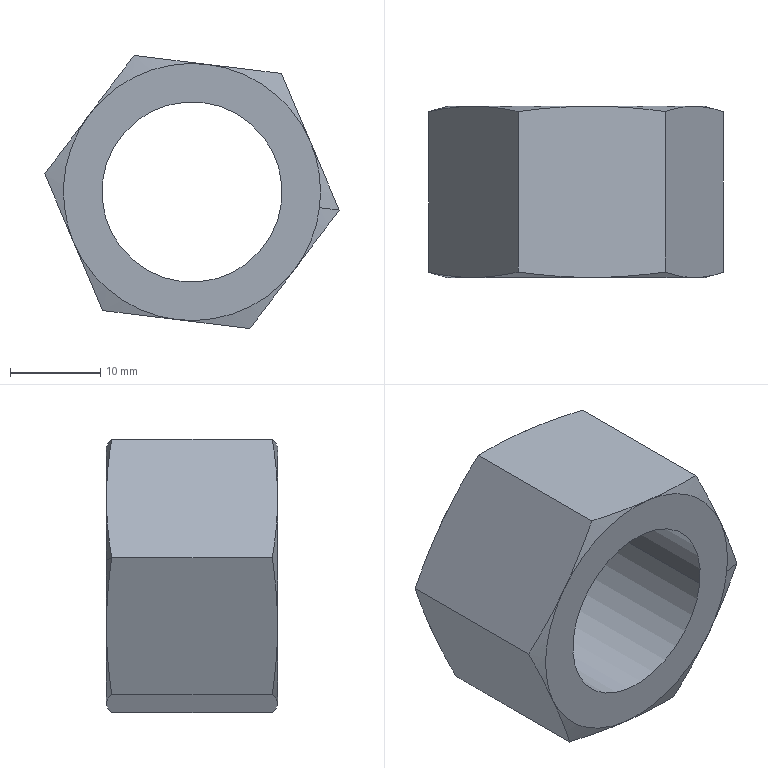Component | SolidWorks | GB_T41-2000HexNutType1C-gradeM20-1 | 1 solid | 24 faces | box 32.7 x 19 x 30.33 mm | volume 7406 mm3 | cone 14 | plane 8 | cylinder 2 | commonest cylinder face diameters 20 x2
STEP:
#1=COLOUR_RGB('',0.7922,0.8196,0.9333);
#2=FILL_AREA_STYLE_COLOUR('',#1);
#3=FILL_AREA_STYLE('',(#2));
#4=SURFACE_STYLE_FILL_AREA(#3);
#5=SURFACE_SIDE_STYLE('',(#4));
#6=SURFACE_STYLE_USAGE(.BOTH.,#5);
#7=PRESENTATION_STYLE_ASSIGNMENT((#6));
#8=CARTESIAN_POINT('',(-12.869,-7.053,5.337));
#9=VERTEX_POINT('',#8);
#10=CARTESIAN_POINT('',(-12.828,-7.053,5.05));
#11=VERTEX_POINT('',#10);
#12=CARTESIAN_POINT('',(-13.386,-7.053,5.118));
#13=DIRECTION('',(-0.,1.,0.));
#14=DIRECTION('',(-0.9925,0.,0.1221));
#15=AXIS2_PLACEMENT_3D('',#12,#13,#14);
#16=CIRCLE('',#15,0.5617);
#17=EDGE_CURVE('',#9,#11,#16,.T.);
#18=ORIENTED_EDGE('',*,*,#17,.T.);
#19=CARTESIAN_POINT('',(-12.742,-7.029,5.039));
#20=VERTEX_POINT('',#19);
#21=CARTESIAN_POINT('',(-12.828,-7.053,5.05));
#22=DIRECTION('',(0.9587,0.2588,-0.1179));
#23=VECTOR('',#22,39.37);
#24=LINE('',#21,#23);
#25=EDGE_CURVE('',#11,#20,#24,.T.);
#26=ORIENTED_EDGE('',*,*,#25,.T.);
#27=CARTESIAN_POINT('',(-12.742,-7.029,5.039));
#28=CARTESIAN_POINT('',(-12.763,-7.036,5.089));
#29=CARTESIAN_POINT('',(-12.784,-7.042,5.138));
#30=CARTESIAN_POINT('',(-12.826,-7.05,5.238));
#31=CARTESIAN_POINT('',(-12.848,-7.053,5.288));
#32=CARTESIAN_POINT('',(-12.869,-7.053,5.337));
#33=B_SPLINE_CURVE_WITH_KNOTS('',3,(#27,#28,#29,#30,#31,#32),.UNSPECIFIED.,.F.,.F.,(4,2,4),(0.00000023,0.004119,0.008238),.UNSPECIFIED.);
#34=EDGE_CURVE('',#20,#9,#33,.T.);
#35=ORIENTED_EDGE('',*,*,#34,.T.);
#36=EDGE_LOOP('',(#18,#26,#35));
#37=FACE_OUTER_BOUND('',#36,.T.);
#38=CARTESIAN_POINT('',(-13.386,-7.053,5.118));
#39=DIRECTION('',(-0.,1.,0.));
#40=DIRECTION('',(0.9925,0.,-0.1221));
#41=AXIS2_PLACEMENT_3D('',#38,#39,#40);
#42=CONICAL_SURFACE('',#41,0.5617,1.309);
#43=ADVANCED_FACE('',(#37),#42,.T.);
#44=CARTESIAN_POINT('',(-13.943,-6.304,5.187));
#45=VERTEX_POINT('',#44);
#46=CARTESIAN_POINT('',(-13.834,-6.304,5.456));
#47=VERTEX_POINT('',#46);
#48=CARTESIAN_POINT('',(-13.386,-6.304,5.118));
#49=DIRECTION('',(-0.,1.,0.));
#50=DIRECTION('',(-0.9925,0.,0.1221));
#51=AXIS2_PLACEMENT_3D('',#48,#49,#50);
#52=CIRCLE('',#51,0.5617);
#53=EDGE_CURVE('',#45,#47,#52,.T.);
#54=ORIENTED_EDGE('',*,*,#53,.F.);
#55=CARTESIAN_POINT('',(-14.03,-6.328,5.197));
#56=VERTEX_POINT('',#55);
#57=CARTESIAN_POINT('',(-13.943,-6.304,5.187));
#58=DIRECTION('',(-0.9587,-0.2588,0.1179));
#59=VECTOR('',#58,39.37);
#60=LINE('',#57,#59);
#61=EDGE_CURVE('',#45,#56,#60,.T.);
#62=ORIENTED_EDGE('',*,*,#61,.T.);
#63=CARTESIAN_POINT('',(-14.03,-6.328,5.197));
#64=CARTESIAN_POINT('',(-13.997,-6.321,5.24));
#65=CARTESIAN_POINT('',(-13.965,-6.315,5.284));
#66=CARTESIAN_POINT('',(-13.899,-6.307,5.37));
#67=CARTESIAN_POINT('',(-13.867,-6.304,5.413));
#68=CARTESIAN_POINT('',(-13.834,-6.304,5.456));
#69=B_SPLINE_CURVE_WITH_KNOTS('',3,(#63,#64,#65,#66,#67,#68),.UNSPECIFIED.,.F.,.F.,(4,2,4),(0.00000023,0.004119,0.008238),.UNSPECIFIED.);
#70=EDGE_CURVE('',#56,#47,#69,.T.);
#71=ORIENTED_EDGE('',*,*,#70,.T.);
#72=EDGE_LOOP('',(#54,#62,#71));
#73=FACE_OUTER_BOUND('',#72,.T.);
#74=CARTESIAN_POINT('',(-13.386,-6.304,5.118));
#75=DIRECTION('',(0.,-1.,-0.));
#76=DIRECTION('',(-0.9925,0.,0.1221));
#77=AXIS2_PLACEMENT_3D('',#74,#75,#76);
#78=CONICAL_SURFACE('',#77,0.5617,1.309);
#79=ADVANCED_FACE('',(#73),#78,.T.);
#80=CARTESIAN_POINT('',(-13.777,-7.053,5.166));
#81=VERTEX_POINT('',#80);
#82=CARTESIAN_POINT('',(-12.995,-7.053,5.07));
#83=VERTEX_POINT('',#82);
#84=CARTESIAN_POINT('',(-13.386,-7.053,5.118));
#85=DIRECTION('',(0.,-1.,-0.));
#86=DIRECTION('',(0.9925,0.,-0.1221));
#87=AXIS2_PLACEMENT_3D('',#84,#85,#86);
#88=CIRCLE('',#87,0.3937);
#89=EDGE_CURVE('',#81,#83,#88,.T.);
#90=ORIENTED_EDGE('',*,*,#89,.T.);
#91=CARTESIAN_POINT('',(-12.995,-6.304,5.07));
#92=VERTEX_POINT('',#91);
#93=CARTESIAN_POINT('',(-12.995,-7.053,5.07));
#94=DIRECTION('',(-0.,1.,0.));
#95=VECTOR('',#94,39.37);
#96=LINE('',#93,#95);
#97=EDGE_CURVE('',#83,#92,#96,.T.);
#98=ORIENTED_EDGE('',*,*,#97,.T.);
#99=CARTESIAN_POINT('',(-13.777,-6.304,5.166));
#100=VERTEX_POINT('',#99);
#101=CARTESIAN_POINT('',(-13.386,-6.304,5.118));
#102=DIRECTION('',(0.,-1.,-0.));
#103=DIRECTION('',(0.9925,0.,-0.1221));
#104=AXIS2_PLACEMENT_3D('',#101,#102,#103);
#105=CIRCLE('',#104,0.3937);
#106=EDGE_CURVE('',#100,#92,#105,.T.);
#107=ORIENTED_EDGE('',*,*,#106,.F.);
#108=CARTESIAN_POINT('',(-13.777,-7.053,5.166));
#109=DIRECTION('',(-0.,1.,0.));
#110=VECTOR('',#109,39.37);
#111=LINE('',#108,#110);
#112=EDGE_CURVE('',#81,#100,#111,.T.);
#113=ORIENTED_EDGE('',*,*,#112,.F.);
#114=EDGE_LOOP('',(#90,#98,#107,#113));
#115=FACE_OUTER_BOUND('',#114,.T.);
#116=CARTESIAN_POINT('',(-13.386,-7.053,5.118));
#117=DIRECTION('',(-0.,1.,0.));
#118=DIRECTION('',(-0.9925,0.,0.1221));
#119=AXIS2_PLACEMENT_3D('',#116,#117,#118);
#120=CYLINDRICAL_SURFACE('',#119,0.3937);
#121=ADVANCED_FACE('',(#115),#120,.F.);
#122=ORIENTED_EDGE('',*,*,#34,.F.);
#123=CARTESIAN_POINT('',(-12.742,-6.328,5.039));
#124=VERTEX_POINT('',#123);
#125=CARTESIAN_POINT('',(-12.742,-7.053,5.039));
#126=DIRECTION('',(-0.,1.,0.));
#127=VECTOR('',#126,39.37);
#128=LINE('',#125,#127);
#129=EDGE_CURVE('',#20,#124,#128,.T.);
#130=ORIENTED_EDGE('',*,*,#129,.T.);
#131=CARTESIAN_POINT('',(-12.869,-6.304,5.337));
#132=VERTEX_POINT('',#131);
#133=CARTESIAN_POINT('',(-12.869,-6.304,5.337));
#134=CARTESIAN_POINT('',(-12.848,-6.304,5.288));
#135=CARTESIAN_POINT('',(-12.826,-6.307,5.238));
#136=CARTESIAN_POINT('',(-12.784,-6.315,5.138));
#137=CARTESIAN_POINT('',(-12.763,-6.321,5.089));
#138=CARTESIAN_POINT('',(-12.742,-6.328,5.039));
#139=B_SPLINE_CURVE_WITH_KNOTS('',3,(#133,#134,#135,#136,#137,#138),.UNSPECIFIED.,.F.,.F.,(4,2,4),(0.008238,0.01236,0.01648),.UNSPECIFIED.);
#140=EDGE_CURVE('',#132,#124,#139,.T.);
#141=ORIENTED_EDGE('',*,*,#140,.F.);
#142=CARTESIAN_POINT('',(-12.995,-6.328,5.636));
#143=VERTEX_POINT('',#142);
#144=CARTESIAN_POINT('',(-12.995,-6.328,5.636));
#145=CARTESIAN_POINT('',(-12.974,-6.321,5.586));
#146=CARTESIAN_POINT('',(-12.953,-6.315,5.537));
#147=CARTESIAN_POINT('',(-12.911,-6.307,5.437));
#148=CARTESIAN_POINT('',(-12.89,-6.304,5.387));
#149=CARTESIAN_POINT('',(-12.869,-6.304,5.337));
#150=B_SPLINE_CURVE_WITH_KNOTS('',3,(#144,#145,#146,#147,#148,#149),.UNSPECIFIED.,.F.,.F.,(4,2,4),(0.00000023,0.004119,0.008238),.UNSPECIFIED.);
#151=EDGE_CURVE('',#143,#132,#150,.T.);
#152=ORIENTED_EDGE('',*,*,#151,.F.);
#153=CARTESIAN_POINT('',(-12.995,-7.029,5.636));
#154=VERTEX_POINT('',#153);
#155=CARTESIAN_POINT('',(-12.995,-7.053,5.636));
#156=DIRECTION('',(-0.,1.,0.));
#157=VECTOR('',#156,39.37);
#158=LINE('',#155,#157);
#159=EDGE_CURVE('',#154,#143,#158,.T.);
#160=ORIENTED_EDGE('',*,*,#159,.F.);
#161=CARTESIAN_POINT('',(-12.869,-7.053,5.337));
#162=CARTESIAN_POINT('',(-12.89,-7.053,5.387));
#163=CARTESIAN_POINT('',(-12.911,-7.05,5.437));
#164=CARTESIAN_POINT('',(-12.953,-7.042,5.537));
#165=CARTESIAN_POINT('',(-12.974,-7.036,5.586));
#166=CARTESIAN_POINT('',(-12.995,-7.029,5.636));
#167=B_SPLINE_CURVE_WITH_KNOTS('',3,(#161,#162,#163,#164,#165,#166),.UNSPECIFIED.,.F.,.F.,(4,2,4),(0.008238,0.01236,0.01648),.UNSPECIFIED.);
#168=EDGE_CURVE('',#9,#154,#167,.T.);
#169=ORIENTED_EDGE('',*,*,#168,.F.);
#170=EDGE_LOOP('',(#122,#130,#141,#152,#160,#169));
#171=FACE_OUTER_BOUND('',#170,.T.);
#172=CARTESIAN_POINT('',(-12.742,-7.053,5.039));
#173=DIRECTION('',(-0.9206,-0.,-0.3905));
#174=DIRECTION('',(0.3905,0.,-0.9206));
#175=AXIS2_PLACEMENT_3D('',#172,#173,#174);
#176=PLANE('',#175);
#177=ADVANCED_FACE('',(#171),#176,.F.);
#178=CARTESIAN_POINT('',(-13.317,-7.053,5.676));
#179=VERTEX_POINT('',#178);
#180=CARTESIAN_POINT('',(-12.995,-7.029,5.636));
#181=CARTESIAN_POINT('',(-13.049,-7.036,5.643));
#182=CARTESIAN_POINT('',(-13.103,-7.042,5.649));
#183=CARTESIAN_POINT('',(-13.21,-7.05,5.662));
#184=CARTESIAN_POINT('',(-13.264,-7.053,5.669));
#185=CARTESIAN_POINT('',(-13.317,-7.053,5.676));
#186=B_SPLINE_CURVE_WITH_KNOTS('',3,(#180,#181,#182,#183,#184,#185),.UNSPECIFIED.,.F.,.F.,(4,2,4),(0.0482,0.05234,0.05648),.UNSPECIFIED.);
#187=EDGE_CURVE('',#154,#179,#186,.T.);
#188=ORIENTED_EDGE('',*,*,#187,.F.);
#189=ORIENTED_EDGE('',*,*,#159,.T.);
#190=CARTESIAN_POINT('',(-13.317,-6.304,5.676));
#191=VERTEX_POINT('',#190);
#192=CARTESIAN_POINT('',(-13.317,-6.304,5.676));
#193=CARTESIAN_POINT('',(-13.264,-6.304,5.669));
#194=CARTESIAN_POINT('',(-13.21,-6.307,5.662));
#195=CARTESIAN_POINT('',(-13.103,-6.315,5.649));
#196=CARTESIAN_POINT('',(-13.049,-6.321,5.643));
#197=CARTESIAN_POINT('',(-12.995,-6.328,5.636));
#198=B_SPLINE_CURVE_WITH_KNOTS('',3,(#192,#193,#194,#195,#196,#197),.UNSPECIFIED.,.F.,.F.,(4,2,4),(0.02237,0.02652,0.03067),.UNSPECIFIED.);
#199=EDGE_CURVE('',#191,#143,#198,.T.);
#200=ORIENTED_EDGE('',*,*,#199,.F.);
#201=CARTESIAN_POINT('',(-13.639,-6.328,5.715));
#202=VERTEX_POINT('',#201);
#203=CARTESIAN_POINT('',(-13.639,-6.328,5.715));
#204=CARTESIAN_POINT('',(-13.586,-6.321,5.709));
#205=CARTESIAN_POINT('',(-13.532,-6.315,5.702));
#206=CARTESIAN_POINT('',(-13.424,-6.307,5.689));
#207=CARTESIAN_POINT('',(-13.371,-6.304,5.682));
#208=CARTESIAN_POINT('',(-13.317,-6.304,5.676));
#209=B_SPLINE_CURVE_WITH_KNOTS('',3,(#203,#204,#205,#206,#207,#208),.UNSPECIFIED.,.F.,.F.,(4,2,4),(0.01409,0.01823,0.02237),.UNSPECIFIED.);
#210=EDGE_CURVE('',#202,#191,#209,.T.);
#211=ORIENTED_EDGE('',*,*,#210,.F.);
#212=CARTESIAN_POINT('',(-13.639,-7.029,5.715));
#213=VERTEX_POINT('',#212);
#214=CARTESIAN_POINT('',(-13.639,-7.053,5.715));
#215=DIRECTION('',(-0.,1.,0.));
#216=VECTOR('',#215,39.37);
#217=LINE('',#214,#216);
#218=EDGE_CURVE('',#213,#202,#217,.T.);
#219=ORIENTED_EDGE('',*,*,#218,.F.);
#220=CARTESIAN_POINT('',(-13.317,-7.053,5.676));
#221=CARTESIAN_POINT('',(-13.371,-7.053,5.682));
#222=CARTESIAN_POINT('',(-13.424,-7.05,5.689));
#223=CARTESIAN_POINT('',(-13.532,-7.042,5.702));
#224=CARTESIAN_POINT('',(-13.586,-7.036,5.709));
#225=CARTESIAN_POINT('',(-13.639,-7.029,5.715));
#226=B_SPLINE_CURVE_WITH_KNOTS('',3,(#220,#221,#222,#223,#224,#225),.UNSPECIFIED.,.F.,.F.,(4,2,4),(0.05648,0.06061,0.06474),.UNSPECIFIED.);
#227=EDGE_CURVE('',#179,#213,#226,.T.);
#228=ORIENTED_EDGE('',*,*,#227,.F.);
#229=EDGE_LOOP('',(#188,#189,#200,#211,#219,#228));
#230=FACE_OUTER_BOUND('',#229,.T.);
#231=CARTESIAN_POINT('',(-12.995,-7.053,5.636));
#232=DIRECTION('',(-0.1221,0.,-0.9925));
#233=DIRECTION('',(0.9925,0.,-0.1221));
#234=AXIS2_PLACEMENT_3D('',#231,#232,#233);
#235=PLANE('',#234);
#236=ADVANCED_FACE('',(#230),#235,.F.);
#237=CARTESIAN_POINT('',(-13.834,-7.053,5.456));
#238=VERTEX_POINT('',#237);
#239=CARTESIAN_POINT('',(-13.639,-7.029,5.715));
#240=CARTESIAN_POINT('',(-13.672,-7.036,5.672));
#241=CARTESIAN_POINT('',(-13.704,-7.042,5.629));
#242=CARTESIAN_POINT('',(-13.769,-7.05,5.543));
#243=CARTESIAN_POINT('',(-13.802,-7.053,5.499));
#244=CARTESIAN_POINT('',(-13.834,-7.053,5.456));
#245=B_SPLINE_CURVE_WITH_KNOTS('',3,(#239,#240,#241,#242,#243,#244),.UNSPECIFIED.,.F.,.F.,(4,2,4),(0.00000023,0.004119,0.008238),.UNSPECIFIED.);
#246=EDGE_CURVE('',#213,#238,#245,.T.);
#247=ORIENTED_EDGE('',*,*,#246,.F.);
#248=ORIENTED_EDGE('',*,*,#218,.T.);
#249=CARTESIAN_POINT('',(-13.834,-6.304,5.456));
#250=CARTESIAN_POINT('',(-13.802,-6.304,5.499));
#251=CARTESIAN_POINT('',(-13.769,-6.307,5.543));
#252=CARTESIAN_POINT('',(-13.704,-6.315,5.629));
#253=CARTESIAN_POINT('',(-13.672,-6.321,5.672));
#254=CARTESIAN_POINT('',(-13.639,-6.328,5.715));
#255=B_SPLINE_CURVE_WITH_KNOTS('',3,(#249,#250,#251,#252,#253,#254),.UNSPECIFIED.,.F.,.F.,(4,2,4),(0.008238,0.01236,0.01648),.UNSPECIFIED.);
#256=EDGE_CURVE('',#47,#202,#255,.T.);
#257=ORIENTED_EDGE('',*,*,#256,.F.);
#258=ORIENTED_EDGE('',*,*,#70,.F.);
#259=CARTESIAN_POINT('',(-14.03,-7.029,5.197));
#260=VERTEX_POINT('',#259);
#261=CARTESIAN_POINT('',(-14.03,-7.053,5.197));
#262=DIRECTION('',(-0.,1.,0.));
#263=VECTOR('',#262,39.37);
#264=LINE('',#261,#263);
#265=EDGE_CURVE('',#260,#56,#264,.T.);
#266=ORIENTED_EDGE('',*,*,#265,.F.);
#267=CARTESIAN_POINT('',(-13.834,-7.053,5.456));
#268=CARTESIAN_POINT('',(-13.867,-7.053,5.413));
#269=CARTESIAN_POINT('',(-13.899,-7.05,5.37));
#270=CARTESIAN_POINT('',(-13.965,-7.042,5.284));
#271=CARTESIAN_POINT('',(-13.997,-7.036,5.24));
#272=CARTESIAN_POINT('',(-14.03,-7.029,5.197));
#273=B_SPLINE_CURVE_WITH_KNOTS('',3,(#267,#268,#269,#270,#271,#272),.UNSPECIFIED.,.F.,.F.,(4,2,4),(0.008238,0.01236,0.01648),.UNSPECIFIED.);
#274=EDGE_CURVE('',#238,#260,#273,.T.);
#275=ORIENTED_EDGE('',*,*,#274,.F.);
#276=EDGE_LOOP('',(#247,#248,#257,#258,#266,#275));
#277=FACE_OUTER_BOUND('',#276,.T.);
#278=CARTESIAN_POINT('',(-13.639,-7.053,5.715));
#279=DIRECTION('',(0.7985,0.,-0.602));
#280=DIRECTION('',(0.602,-0.,0.7985));
#281=AXIS2_PLACEMENT_3D('',#278,#279,#280);
#282=PLANE('',#281);
#283=ADVANCED_FACE('',(#277),#282,.F.);
#284=CARTESIAN_POINT('',(-13.903,-7.053,4.899));
#285=VERTEX_POINT('',#284);
#286=CARTESIAN_POINT('',(-14.03,-7.029,5.197));
#287=CARTESIAN_POINT('',(-14.008,-7.036,5.148));
#288=CARTESIAN_POINT('',(-13.987,-7.042,5.098));
#289=CARTESIAN_POINT('',(-13.945,-7.05,4.998));
#290=CARTESIAN_POINT('',(-13.924,-7.053,4.948));
#291=CARTESIAN_POINT('',(-13.903,-7.053,4.899));
#292=B_SPLINE_CURVE_WITH_KNOTS('',3,(#286,#287,#288,#289,#290,#291),.UNSPECIFIED.,.F.,.F.,(4,2,4),(0.00000023,0.004119,0.008238),.UNSPECIFIED.);
#293=EDGE_CURVE('',#260,#285,#292,.T.);
#294=ORIENTED_EDGE('',*,*,#293,.F.);
#295=ORIENTED_EDGE('',*,*,#265,.T.);
#296=CARTESIAN_POINT('',(-13.903,-6.304,4.899));
#297=VERTEX_POINT('',#296);
#298=CARTESIAN_POINT('',(-13.903,-6.304,4.899));
#299=CARTESIAN_POINT('',(-13.924,-6.304,4.948));
#300=CARTESIAN_POINT('',(-13.945,-6.307,4.998));
#301=CARTESIAN_POINT('',(-13.987,-6.315,5.098));
#302=CARTESIAN_POINT('',(-14.008,-6.321,5.148));
#303=CARTESIAN_POINT('',(-14.03,-6.328,5.197));
#304=B_SPLINE_CURVE_WITH_KNOTS('',3,(#298,#299,#300,#301,#302,#303),.UNSPECIFIED.,.F.,.F.,(4,2,4),(0.008238,0.01236,0.01648),.UNSPECIFIED.);
#305=EDGE_CURVE('',#297,#56,#304,.T.);
#306=ORIENTED_EDGE('',*,*,#305,.F.);
#307=CARTESIAN_POINT('',(-13.776,-6.328,4.6));
#308=VERTEX_POINT('',#307);
#309=CARTESIAN_POINT('',(-13.776,-6.328,4.6));
#310=CARTESIAN_POINT('',(-13.797,-6.321,4.65));
#311=CARTESIAN_POINT('',(-13.819,-6.315,4.7));
#312=CARTESIAN_POINT('',(-13.861,-6.307,4.799));
#313=CARTESIAN_POINT('',(-13.882,-6.304,4.849));
#314=CARTESIAN_POINT('',(-13.903,-6.304,4.899));
#315=B_SPLINE_CURVE_WITH_KNOTS('',3,(#309,#310,#311,#312,#313,#314),.UNSPECIFIED.,.F.,.F.,(4,2,4),(0.00000023,0.004119,0.008238),.UNSPECIFIED.);
#316=EDGE_CURVE('',#308,#297,#315,.T.);
#317=ORIENTED_EDGE('',*,*,#316,.F.);
#318=CARTESIAN_POINT('',(-13.776,-7.029,4.6));
#319=VERTEX_POINT('',#318);
#320=CARTESIAN_POINT('',(-13.776,-7.053,4.6));
#321=DIRECTION('',(-0.,1.,0.));
#322=VECTOR('',#321,39.37);
#323=LINE('',#320,#322);
#324=EDGE_CURVE('',#319,#308,#323,.T.);
#325=ORIENTED_EDGE('',*,*,#324,.F.);
#326=CARTESIAN_POINT('',(-13.903,-7.053,4.899));
#327=CARTESIAN_POINT('',(-13.882,-7.053,4.849));
#328=CARTESIAN_POINT('',(-13.861,-7.05,4.799));
#329=CARTESIAN_POINT('',(-13.819,-7.042,4.7));
#330=CARTESIAN_POINT('',(-13.797,-7.036,4.65));
#331=CARTESIAN_POINT('',(-13.776,-7.029,4.6));
#332=B_SPLINE_CURVE_WITH_KNOTS('',3,(#326,#327,#328,#329,#330,#331),.UNSPECIFIED.,.F.,.F.,(4,2,4),(0.008238,0.01236,0.01648),.UNSPECIFIED.);
#333=EDGE_CURVE('',#285,#319,#332,.T.);
#334=ORIENTED_EDGE('',*,*,#333,.F.);
#335=EDGE_LOOP('',(#294,#295,#306,#317,#325,#334));
#336=FACE_OUTER_BOUND('',#335,.T.);
#337=CARTESIAN_POINT('',(-14.03,-7.053,5.197));
#338=DIRECTION('',(0.9206,0.,0.3905));
#339=DIRECTION('',(-0.3905,-0.,0.9206));
#340=AXIS2_PLACEMENT_3D('',#337,#338,#339);
#341=PLANE('',#340);
#342=ADVANCED_FACE('',(#336),#341,.F.);
#343=CARTESIAN_POINT('',(-13.454,-7.053,4.561));
#344=VERTEX_POINT('',#343);
#345=CARTESIAN_POINT('',(-13.776,-7.029,4.6));
#346=CARTESIAN_POINT('',(-13.723,-7.036,4.594));
#347=CARTESIAN_POINT('',(-13.669,-7.042,4.587));
#348=CARTESIAN_POINT('',(-13.562,-7.05,4.574));
#349=CARTESIAN_POINT('',(-13.508,-7.053,4.567));
#350=CARTESIAN_POINT('',(-13.454,-7.053,4.561));
#351=B_SPLINE_CURVE_WITH_KNOTS('',3,(#345,#346,#347,#348,#349,#350),.UNSPECIFIED.,.F.,.F.,(4,2,4),(0.01409,0.01823,0.02237),.UNSPECIFIED.);
#352=EDGE_CURVE('',#319,#344,#351,.T.);
#353=ORIENTED_EDGE('',*,*,#352,.F.);
#354=ORIENTED_EDGE('',*,*,#324,.T.);
#355=CARTESIAN_POINT('',(-13.454,-6.304,4.561));
#356=VERTEX_POINT('',#355);
#357=CARTESIAN_POINT('',(-13.454,-6.304,4.561));
#358=CARTESIAN_POINT('',(-13.508,-6.304,4.567));
#359=CARTESIAN_POINT('',(-13.562,-6.307,4.574));
#360=CARTESIAN_POINT('',(-13.669,-6.315,4.587));
#361=CARTESIAN_POINT('',(-13.723,-6.321,4.594));
#362=CARTESIAN_POINT('',(-13.776,-6.328,4.6));
#363=B_SPLINE_CURVE_WITH_KNOTS('',3,(#357,#358,#359,#360,#361,#362),.UNSPECIFIED.,.F.,.F.,(4,2,4),(0.05648,0.06061,0.06474),.UNSPECIFIED.);
#364=EDGE_CURVE('',#356,#308,#363,.T.);
#365=ORIENTED_EDGE('',*,*,#364,.F.);
#366=CARTESIAN_POINT('',(-13.133,-6.328,4.521));
#367=VERTEX_POINT('',#366);
#368=CARTESIAN_POINT('',(-13.133,-6.328,4.521));
#369=CARTESIAN_POINT('',(-13.186,-6.321,4.528));
#370=CARTESIAN_POINT('',(-13.24,-6.315,4.534));
#371=CARTESIAN_POINT('',(-13.347,-6.307,4.547));
#372=CARTESIAN_POINT('',(-13.401,-6.304,4.554));
#373=CARTESIAN_POINT('',(-13.454,-6.304,4.561));
#374=B_SPLINE_CURVE_WITH_KNOTS('',3,(#368,#369,#370,#371,#372,#373),.UNSPECIFIED.,.F.,.F.,(4,2,4),(0.0482,0.05234,0.05648),.UNSPECIFIED.);
#375=EDGE_CURVE('',#367,#356,#374,.T.);
#376=ORIENTED_EDGE('',*,*,#375,.F.);
#377=CARTESIAN_POINT('',(-13.133,-7.029,4.521));
#378=VERTEX_POINT('',#377);
#379=CARTESIAN_POINT('',(-13.133,-7.053,4.521));
#380=DIRECTION('',(-0.,1.,0.));
#381=VECTOR('',#380,39.37);
#382=LINE('',#379,#381);
#383=EDGE_CURVE('',#378,#367,#382,.T.);
#384=ORIENTED_EDGE('',*,*,#383,.F.);
#385=CARTESIAN_POINT('',(-13.454,-7.053,4.561));
#386=CARTESIAN_POINT('',(-13.401,-7.053,4.554));
#387=CARTESIAN_POINT('',(-13.347,-7.05,4.547));
#388=CARTESIAN_POINT('',(-13.24,-7.042,4.534));
#389=CARTESIAN_POINT('',(-13.186,-7.036,4.528));
#390=CARTESIAN_POINT('',(-13.133,-7.029,4.521));
#391=B_SPLINE_CURVE_WITH_KNOTS('',3,(#385,#386,#387,#388,#389,#390),.UNSPECIFIED.,.F.,.F.,(4,2,4),(0.02237,0.02652,0.03067),.UNSPECIFIED.);
#392=EDGE_CURVE('',#344,#378,#391,.T.);
#393=ORIENTED_EDGE('',*,*,#392,.F.);
#394=EDGE_LOOP('',(#353,#354,#365,#376,#384,#393));
#395=FACE_OUTER_BOUND('',#394,.T.);
#396=CARTESIAN_POINT('',(-13.776,-7.053,4.6));
#397=DIRECTION('',(0.1221,-0.,0.9925));
#398=DIRECTION('',(-0.9925,-0.,0.1221));
#399=AXIS2_PLACEMENT_3D('',#396,#397,#398);
#400=PLANE('',#399);
#401=ADVANCED_FACE('',(#395),#400,.F.);
#402=CARTESIAN_POINT('',(-12.937,-7.053,4.78));
#403=VERTEX_POINT('',#402);
#404=CARTESIAN_POINT('',(-13.133,-7.029,4.521));
#405=CARTESIAN_POINT('',(-13.1,-7.036,4.564));
#406=CARTESIAN_POINT('',(-13.067,-7.042,4.607));
#407=CARTESIAN_POINT('',(-13.002,-7.05,4.694));
#408=CARTESIAN_POINT('',(-12.97,-7.053,4.737));
#409=CARTESIAN_POINT('',(-12.937,-7.053,4.78));
#410=B_SPLINE_CURVE_WITH_KNOTS('',3,(#404,#405,#406,#407,#408,#409),.UNSPECIFIED.,.F.,.F.,(4,2,4),(0.00000023,0.004119,0.008238),.UNSPECIFIED.);
#411=EDGE_CURVE('',#378,#403,#410,.T.);
#412=ORIENTED_EDGE('',*,*,#411,.F.);
#413=ORIENTED_EDGE('',*,*,#383,.T.);
#414=CARTESIAN_POINT('',(-12.937,-6.304,4.78));
#415=VERTEX_POINT('',#414);
#416=CARTESIAN_POINT('',(-12.937,-6.304,4.78));
#417=CARTESIAN_POINT('',(-12.97,-6.304,4.737));
#418=CARTESIAN_POINT('',(-13.002,-6.307,4.694));
#419=CARTESIAN_POINT('',(-13.067,-6.315,4.607));
#420=CARTESIAN_POINT('',(-13.1,-6.321,4.564));
#421=CARTESIAN_POINT('',(-13.133,-6.328,4.521));
#422=B_SPLINE_CURVE_WITH_KNOTS('',3,(#416,#417,#418,#419,#420,#421),.UNSPECIFIED.,.F.,.F.,(4,2,4),(0.008238,0.01236,0.01648),.UNSPECIFIED.);
#423=EDGE_CURVE('',#415,#367,#422,.T.);
#424=ORIENTED_EDGE('',*,*,#423,.F.);
#425=CARTESIAN_POINT('',(-12.742,-6.328,5.039));
#426=CARTESIAN_POINT('',(-12.775,-6.321,4.996));
#427=CARTESIAN_POINT('',(-12.807,-6.315,4.953));
#428=CARTESIAN_POINT('',(-12.872,-6.307,4.866));
#429=CARTESIAN_POINT('',(-12.905,-6.304,4.823));
#430=CARTESIAN_POINT('',(-12.937,-6.304,4.78));
#431=B_SPLINE_CURVE_WITH_KNOTS('',3,(#425,#426,#427,#428,#429,#430),.UNSPECIFIED.,.F.,.F.,(4,2,4),(0.00000023,0.004119,0.008238),.UNSPECIFIED.);
#432=EDGE_CURVE('',#124,#415,#431,.T.);
#433=ORIENTED_EDGE('',*,*,#432,.F.);
#434=ORIENTED_EDGE('',*,*,#129,.F.);
#435=CARTESIAN_POINT('',(-12.937,-7.053,4.78));
#436=CARTESIAN_POINT('',(-12.905,-7.053,4.823));
#437=CARTESIAN_POINT('',(-12.872,-7.05,4.866));
#438=CARTESIAN_POINT('',(-12.807,-7.042,4.953));
#439=CARTESIAN_POINT('',(-12.775,-7.036,4.996));
#440=CARTESIAN_POINT('',(-12.742,-7.029,5.039));
#441=B_SPLINE_CURVE_WITH_KNOTS('',3,(#435,#436,#437,#438,#439,#440),.UNSPECIFIED.,.F.,.F.,(4,2,4),(0.008238,0.01236,0.01648),.UNSPECIFIED.);
#442=EDGE_CURVE('',#403,#20,#441,.T.);
#443=ORIENTED_EDGE('',*,*,#442,.F.);
#444=EDGE_LOOP('',(#412,#413,#424,#433,#434,#443));
#445=FACE_OUTER_BOUND('',#444,.T.);
#446=CARTESIAN_POINT('',(-13.133,-7.053,4.521));
#447=DIRECTION('',(-0.7985,-0.,0.602));
#448=DIRECTION('',(-0.602,0.,-0.7985));
#449=AXIS2_PLACEMENT_3D('',#446,#447,#448);
#450=PLANE('',#449);
#451=ADVANCED_FACE('',(#445),#450,.F.);
#452=ORIENTED_EDGE('',*,*,#89,.F.);
#453=CARTESIAN_POINT('',(-13.386,-7.053,5.118));
#454=DIRECTION('',(0.,-1.,-0.));
#455=DIRECTION('',(0.9925,0.,-0.1221));
#456=AXIS2_PLACEMENT_3D('',#453,#454,#455);
#457=CIRCLE('',#456,0.3937);
#458=EDGE_CURVE('',#83,#81,#457,.T.);
#459=ORIENTED_EDGE('',*,*,#458,.F.);
#460=EDGE_LOOP('',(#452,#459));
#461=FACE_BOUND('',#460,.T.);
#462=CARTESIAN_POINT('',(-13.386,-7.053,5.118));
#463=DIRECTION('',(-0.,1.,0.));
#464=DIRECTION('',(-0.9925,0.,0.1221));
#465=AXIS2_PLACEMENT_3D('',#462,#463,#464);
#466=CIRCLE('',#465,0.5617);
#467=EDGE_CURVE('',#238,#179,#466,.T.);
#468=ORIENTED_EDGE('',*,*,#467,.F.);
#469=CARTESIAN_POINT('',(-13.386,-7.053,5.118));
#470=DIRECTION('',(-0.,1.,0.));
#471=DIRECTION('',(-0.9925,0.,0.1221));
#472=AXIS2_PLACEMENT_3D('',#469,#470,#471);
#473=CIRCLE('',#472,0.5617);
#474=EDGE_CURVE('',#285,#238,#473,.T.);
#475=ORIENTED_EDGE('',*,*,#474,.F.);
#476=CARTESIAN_POINT('',(-13.386,-7.053,5.118));
#477=DIRECTION('',(-0.,1.,0.));
#478=DIRECTION('',(-0.9925,0.,0.1221));
#479=AXIS2_PLACEMENT_3D('',#476,#477,#478);
#480=CIRCLE('',#479,0.5617);
#481=EDGE_CURVE('',#344,#285,#480,.T.);
#482=ORIENTED_EDGE('',*,*,#481,.F.);
#483=CARTESIAN_POINT('',(-13.386,-7.053,5.118));
#484=DIRECTION('',(-0.,1.,0.));
#485=DIRECTION('',(-0.9925,0.,0.1221));
#486=AXIS2_PLACEMENT_3D('',#483,#484,#485);
#487=CIRCLE('',#486,0.5617);
#488=EDGE_CURVE('',#403,#344,#487,.T.);
#489=ORIENTED_EDGE('',*,*,#488,.F.);
#490=CARTESIAN_POINT('',(-13.386,-7.053,5.118));
#491=DIRECTION('',(-0.,1.,0.));
#492=DIRECTION('',(-0.9925,0.,0.1221));
#493=AXIS2_PLACEMENT_3D('',#490,#491,#492);
#494=CIRCLE('',#493,0.5617);
#495=EDGE_CURVE('',#11,#403,#494,.T.);
#496=ORIENTED_EDGE('',*,*,#495,.F.);
#497=ORIENTED_EDGE('',*,*,#17,.F.);
#498=CARTESIAN_POINT('',(-13.386,-7.053,5.118));
#499=DIRECTION('',(0.,-1.,-0.));
#500=DIRECTION('',(0.9925,0.,-0.1221));
#501=AXIS2_PLACEMENT_3D('',#498,#499,#500);
#502=CIRCLE('',#501,0.5617);
#503=EDGE_CURVE('',#9,#179,#502,.T.);
#504=ORIENTED_EDGE('',*,*,#503,.T.);
#505=EDGE_LOOP('',(#468,#475,#482,#489,#496,#497,#504));
#506=FACE_OUTER_BOUND('',#505,.T.);
#507=CARTESIAN_POINT('',(-12.489,-7.053,4.442));
#508=DIRECTION('',(-0.,1.,0.));
#509=DIRECTION('',(-0.9925,-0.,0.1221));
#510=AXIS2_PLACEMENT_3D('',#507,#508,#509);
#511=PLANE('',#510);
#512=ADVANCED_FACE('',(#461,#506),#511,.F.);
#513=ORIENTED_EDGE('',*,*,#106,.T.);
#514=CARTESIAN_POINT('',(-13.386,-6.304,5.118));
#515=DIRECTION('',(0.,-1.,-0.));
#516=DIRECTION('',(0.9925,0.,-0.1221));
#517=AXIS2_PLACEMENT_3D('',#514,#515,#516);
#518=CIRCLE('',#517,0.3937);
#519=EDGE_CURVE('',#92,#100,#518,.T.);
#520=ORIENTED_EDGE('',*,*,#519,.T.);
#521=EDGE_LOOP('',(#513,#520));
#522=FACE_BOUND('',#521,.T.);
#523=CARTESIAN_POINT('',(-13.386,-6.304,5.118));
#524=DIRECTION('',(-0.,1.,0.));
#525=DIRECTION('',(-0.9925,0.,0.1221));
#526=AXIS2_PLACEMENT_3D('',#523,#524,#525);
#527=CIRCLE('',#526,0.5617);
#528=EDGE_CURVE('',#297,#45,#527,.T.);
#529=ORIENTED_EDGE('',*,*,#528,.T.);
#530=ORIENTED_EDGE('',*,*,#53,.T.);
#531=CARTESIAN_POINT('',(-13.386,-6.304,5.118));
#532=DIRECTION('',(-0.,1.,0.));
#533=DIRECTION('',(-0.9925,0.,0.1221));
#534=AXIS2_PLACEMENT_3D('',#531,#532,#533);
#535=CIRCLE('',#534,0.5617);
#536=EDGE_CURVE('',#47,#191,#535,.T.);
#537=ORIENTED_EDGE('',*,*,#536,.T.);
#538=CARTESIAN_POINT('',(-13.386,-6.304,5.118));
#539=DIRECTION('',(-0.,1.,0.));
#540=DIRECTION('',(-0.9925,0.,0.1221));
#541=AXIS2_PLACEMENT_3D('',#538,#539,#540);
#542=CIRCLE('',#541,0.5617);
#543=EDGE_CURVE('',#191,#132,#542,.T.);
#544=ORIENTED_EDGE('',*,*,#543,.T.);
#545=CARTESIAN_POINT('',(-13.386,-6.304,5.118));
#546=DIRECTION('',(-0.,1.,0.));
#547=DIRECTION('',(-0.9925,0.,0.1221));
#548=AXIS2_PLACEMENT_3D('',#545,#546,#547);
#549=CIRCLE('',#548,0.5617);
#550=EDGE_CURVE('',#132,#415,#549,.T.);
#551=ORIENTED_EDGE('',*,*,#550,.T.);
#552=CARTESIAN_POINT('',(-13.386,-6.304,5.118));
#553=DIRECTION('',(-0.,1.,0.));
#554=DIRECTION('',(-0.9925,0.,0.1221));
#555=AXIS2_PLACEMENT_3D('',#552,#553,#554);
#556=CIRCLE('',#555,0.5617);
#557=EDGE_CURVE('',#415,#356,#556,.T.);
#558=ORIENTED_EDGE('',*,*,#557,.T.);
#559=CARTESIAN_POINT('',(-13.386,-6.304,5.118));
#560=DIRECTION('',(-0.,1.,0.));
#561=DIRECTION('',(-0.9925,0.,0.1221));
#562=AXIS2_PLACEMENT_3D('',#559,#560,#561);
#563=CIRCLE('',#562,0.5617);
#564=EDGE_CURVE('',#356,#297,#563,.T.);
#565=ORIENTED_EDGE('',*,*,#564,.T.);
#566=EDGE_LOOP('',(#529,#530,#537,#544,#551,#558,#565));
#567=FACE_OUTER_BOUND('',#566,.T.);
#568=CARTESIAN_POINT('',(-12.489,-6.304,4.442));
#569=DIRECTION('',(-0.,1.,0.));
#570=DIRECTION('',(-0.9925,-0.,0.1221));
#571=AXIS2_PLACEMENT_3D('',#568,#569,#570);
#572=PLANE('',#571);
#573=ADVANCED_FACE('',(#522,#567),#572,.T.);
#574=ORIENTED_EDGE('',*,*,#97,.F.);
#575=ORIENTED_EDGE('',*,*,#458,.T.);
#576=ORIENTED_EDGE('',*,*,#112,.T.);
#577=ORIENTED_EDGE('',*,*,#519,.F.);
#578=EDGE_LOOP('',(#574,#575,#576,#577));
#579=FACE_OUTER_BOUND('',#578,.T.);
#580=CARTESIAN_POINT('',(-13.386,-7.053,5.118));
#581=DIRECTION('',(-0.,1.,0.));
#582=DIRECTION('',(-0.9925,0.,0.1221));
#583=AXIS2_PLACEMENT_3D('',#580,#581,#582);
#584=CYLINDRICAL_SURFACE('',#583,0.3937);
#585=ADVANCED_FACE('',(#579),#584,.F.);
#586=ORIENTED_EDGE('',*,*,#375,.T.);
#587=ORIENTED_EDGE('',*,*,#557,.F.);
#588=ORIENTED_EDGE('',*,*,#423,.T.);
#589=EDGE_LOOP('',(#586,#587,#588));
#590=FACE_OUTER_BOUND('',#589,.T.);
#591=CARTESIAN_POINT('',(-13.386,-6.304,5.118));
#592=DIRECTION('',(0.,-1.,-0.));
#593=DIRECTION('',(-0.9925,0.,0.1221));
#594=AXIS2_PLACEMENT_3D('',#591,#592,#593);
#595=CONICAL_SURFACE('',#594,0.5617,1.309);
#596=ADVANCED_FACE('',(#590),#595,.T.);
#597=ORIENTED_EDGE('',*,*,#140,.T.);
#598=ORIENTED_EDGE('',*,*,#432,.T.);
#599=ORIENTED_EDGE('',*,*,#550,.F.);
#600=EDGE_LOOP('',(#597,#598,#599));
#601=FACE_OUTER_BOUND('',#600,.T.);
#602=CARTESIAN_POINT('',(-13.386,-6.304,5.118));
#603=DIRECTION('',(0.,-1.,-0.));
#604=DIRECTION('',(-0.9925,0.,0.1221));
#605=AXIS2_PLACEMENT_3D('',#602,#603,#604);
#606=CONICAL_SURFACE('',#605,0.5617,1.309);
#607=ADVANCED_FACE('',(#601),#606,.T.);
#608=ORIENTED_EDGE('',*,*,#316,.T.);
#609=ORIENTED_EDGE('',*,*,#564,.F.);
#610=ORIENTED_EDGE('',*,*,#364,.T.);
#611=EDGE_LOOP('',(#608,#609,#610));
#612=FACE_OUTER_BOUND('',#611,.T.);
#613=CARTESIAN_POINT('',(-13.386,-6.304,5.118));
#614=DIRECTION('',(0.,-1.,-0.));
#615=DIRECTION('',(-0.9925,0.,0.1221));
#616=AXIS2_PLACEMENT_3D('',#613,#614,#615);
#617=CONICAL_SURFACE('',#616,0.5617,1.309);
#618=ADVANCED_FACE('',(#612),#617,.T.);
#619=ORIENTED_EDGE('',*,*,#61,.F.);
#620=ORIENTED_EDGE('',*,*,#528,.F.);
#621=ORIENTED_EDGE('',*,*,#305,.T.);
#622=EDGE_LOOP('',(#619,#620,#621));
#623=FACE_OUTER_BOUND('',#622,.T.);
#624=CARTESIAN_POINT('',(-13.386,-6.304,5.118));
#625=DIRECTION('',(0.,-1.,-0.));
#626=DIRECTION('',(-0.9925,0.,0.1221));
#627=AXIS2_PLACEMENT_3D('',#624,#625,#626);
#628=CONICAL_SURFACE('',#627,0.5617,1.309);
#629=ADVANCED_FACE('',(#623),#628,.T.);
#630=ORIENTED_EDGE('',*,*,#256,.T.);
#631=ORIENTED_EDGE('',*,*,#210,.T.);
#632=ORIENTED_EDGE('',*,*,#536,.F.);
#633=EDGE_LOOP('',(#630,#631,#632));
#634=FACE_OUTER_BOUND('',#633,.T.);
#635=CARTESIAN_POINT('',(-13.386,-6.304,5.118));
#636=DIRECTION('',(0.,-1.,-0.));
#637=DIRECTION('',(-0.9925,0.,0.1221));
#638=AXIS2_PLACEMENT_3D('',#635,#636,#637);
#639=CONICAL_SURFACE('',#638,0.5617,1.309);
#640=ADVANCED_FACE('',(#634),#639,.T.);
#641=ORIENTED_EDGE('',*,*,#199,.T.);
#642=ORIENTED_EDGE('',*,*,#151,.T.);
#643=ORIENTED_EDGE('',*,*,#543,.F.);
#644=EDGE_LOOP('',(#641,#642,#643));
#645=FACE_OUTER_BOUND('',#644,.T.);
#646=CARTESIAN_POINT('',(-13.386,-6.304,5.118));
#647=DIRECTION('',(0.,-1.,-0.));
#648=DIRECTION('',(-0.9925,0.,0.1221));
#649=AXIS2_PLACEMENT_3D('',#646,#647,#648);
#650=CONICAL_SURFACE('',#649,0.5617,1.309);
#651=ADVANCED_FACE('',(#645),#650,.T.);
#652=ORIENTED_EDGE('',*,*,#274,.T.);
#653=ORIENTED_EDGE('',*,*,#293,.T.);
#654=ORIENTED_EDGE('',*,*,#474,.T.);
#655=EDGE_LOOP('',(#652,#653,#654));
#656=FACE_OUTER_BOUND('',#655,.T.);
#657=CARTESIAN_POINT('',(-13.386,-7.053,5.118));
#658=DIRECTION('',(-0.,1.,0.));
#659=DIRECTION('',(0.9925,0.,-0.1221));
#660=AXIS2_PLACEMENT_3D('',#657,#658,#659);
#661=CONICAL_SURFACE('',#660,0.5617,1.309);
#662=ADVANCED_FACE('',(#656),#661,.T.);
#663=ORIENTED_EDGE('',*,*,#333,.T.);
#664=ORIENTED_EDGE('',*,*,#352,.T.);
#665=ORIENTED_EDGE('',*,*,#481,.T.);
#666=EDGE_LOOP('',(#663,#664,#665));
#667=FACE_OUTER_BOUND('',#666,.T.);
#668=CARTESIAN_POINT('',(-13.386,-7.053,5.118));
#669=DIRECTION('',(-0.,1.,0.));
#670=DIRECTION('',(0.9925,0.,-0.1221));
#671=AXIS2_PLACEMENT_3D('',#668,#669,#670);
#672=CONICAL_SURFACE('',#671,0.5617,1.309);
#673=ADVANCED_FACE('',(#667),#672,.T.);
#674=ORIENTED_EDGE('',*,*,#392,.T.);
#675=ORIENTED_EDGE('',*,*,#411,.T.);
#676=ORIENTED_EDGE('',*,*,#488,.T.);
#677=EDGE_LOOP('',(#674,#675,#676));
#678=FACE_OUTER_BOUND('',#677,.T.);
#679=CARTESIAN_POINT('',(-13.386,-7.053,5.118));
#680=DIRECTION('',(-0.,1.,0.));
#681=DIRECTION('',(0.9925,0.,-0.1221));
#682=AXIS2_PLACEMENT_3D('',#679,#680,#681);
#683=CONICAL_SURFACE('',#682,0.5617,1.309);
#684=ADVANCED_FACE('',(#678),#683,.T.);
#685=ORIENTED_EDGE('',*,*,#25,.F.);
#686=ORIENTED_EDGE('',*,*,#495,.T.);
#687=ORIENTED_EDGE('',*,*,#442,.T.);
#688=EDGE_LOOP('',(#685,#686,#687));
#689=FACE_OUTER_BOUND('',#688,.T.);
#690=CARTESIAN_POINT('',(-13.386,-7.053,5.118));
#691=DIRECTION('',(-0.,1.,0.));
#692=DIRECTION('',(0.9925,0.,-0.1221));
#693=AXIS2_PLACEMENT_3D('',#690,#691,#692);
#694=CONICAL_SURFACE('',#693,0.5617,1.309);
#695=ADVANCED_FACE('',(#689),#694,.T.);
#696=ORIENTED_EDGE('',*,*,#168,.T.);
#697=ORIENTED_EDGE('',*,*,#187,.T.);
#698=ORIENTED_EDGE('',*,*,#503,.F.);
#699=EDGE_LOOP('',(#696,#697,#698));
#700=FACE_OUTER_BOUND('',#699,.T.);
#701=CARTESIAN_POINT('',(-13.386,-7.053,5.118));
#702=DIRECTION('',(-0.,1.,0.));
#703=DIRECTION('',(0.9925,0.,-0.1221));
#704=AXIS2_PLACEMENT_3D('',#701,#702,#703);
#705=CONICAL_SURFACE('',#704,0.5617,1.309);
#706=ADVANCED_FACE('',(#700),#705,.T.);
#707=ORIENTED_EDGE('',*,*,#227,.T.);
#708=ORIENTED_EDGE('',*,*,#246,.T.);
#709=ORIENTED_EDGE('',*,*,#467,.T.);
#710=EDGE_LOOP('',(#707,#708,#709));
#711=FACE_OUTER_BOUND('',#710,.T.);
#712=CARTESIAN_POINT('',(-13.386,-7.053,5.118));
#713=DIRECTION('',(-0.,1.,0.));
#714=DIRECTION('',(0.9925,0.,-0.1221));
#715=AXIS2_PLACEMENT_3D('',#712,#713,#714);
#716=CONICAL_SURFACE('',#715,0.5617,1.309);
#717=ADVANCED_FACE('',(#711),#716,.T.);
#718=CLOSED_SHELL('',(#43,#79,#121,#177,#236,#283,#342,#401,#451,#512,#573,#585,#596,#607,#618,#629,#640,#651,#662,#673,#684,#695,#706,#717));
#719=MANIFOLD_SOLID_BREP('',#718);
#720=STYLED_ITEM('',(#7),#719);
#721=(LENGTH_UNIT()NAMED_UNIT(*)SI_UNIT($,.METRE.));
#722=LENGTH_MEASURE_WITH_UNIT(LENGTH_MEASURE(0.0254),#721);
#723=DIMENSIONAL_EXPONENTS(1.,0.,0.,0.,0.,0.,0.);
#724=(CONVERSION_BASED_UNIT('',#722)LENGTH_UNIT()NAMED_UNIT(#723));
#725=UNCERTAINTY_MEASURE_WITH_UNIT(LENGTH_MEASURE(0.00001),#724,'','');
#726=(NAMED_UNIT(*)PLANE_ANGLE_UNIT()SI_UNIT($,.RADIAN.));
#727=(NAMED_UNIT(*)SI_UNIT($,.STERADIAN.)SOLID_ANGLE_UNIT());
#728=(GEOMETRIC_REPRESENTATION_CONTEXT(3)GLOBAL_UNCERTAINTY_ASSIGNED_CONTEXT((#725))GLOBAL_UNIT_ASSIGNED_CONTEXT((#724,#726,#727))REPRESENTATION_CONTEXT('',''));
#729=MECHANICAL_DESIGN_GEOMETRIC_PRESENTATION_REPRESENTATION('',(#720),#728);
#730=PRESENTATION_LAYER_ASSIGNMENT('','',(#720));
#731=CARTESIAN_POINT('',(0.,0.,0.));
#732=DIRECTION('',(0.,0.,1.));
#733=DIRECTION('',(1.,0.,0.));
#734=AXIS2_PLACEMENT_3D('',#731,#732,#733);
#735=(LENGTH_UNIT()NAMED_UNIT(*)SI_UNIT($,.METRE.));
#736=LENGTH_MEASURE_WITH_UNIT(LENGTH_MEASURE(0.0254),#735);
#737=DIMENSIONAL_EXPONENTS(1.,0.,0.,0.,0.,0.,0.);
#738=(CONVERSION_BASED_UNIT('',#736)LENGTH_UNIT()NAMED_UNIT(#737));
#739=UNCERTAINTY_MEASURE_WITH_UNIT(LENGTH_MEASURE(0.00001),#738,'','');
#740=(NAMED_UNIT(*)PLANE_ANGLE_UNIT()SI_UNIT($,.RADIAN.));
#741=(NAMED_UNIT(*)SI_UNIT($,.STERADIAN.)SOLID_ANGLE_UNIT());
#742=(GEOMETRIC_REPRESENTATION_CONTEXT(3)GLOBAL_UNCERTAINTY_ASSIGNED_CONTEXT((#739))GLOBAL_UNIT_ASSIGNED_CONTEXT((#738,#740,#741))REPRESENTATION_CONTEXT('',''));
#743=ADVANCED_BREP_SHAPE_REPRESENTATION('',(#719,#734),#742);